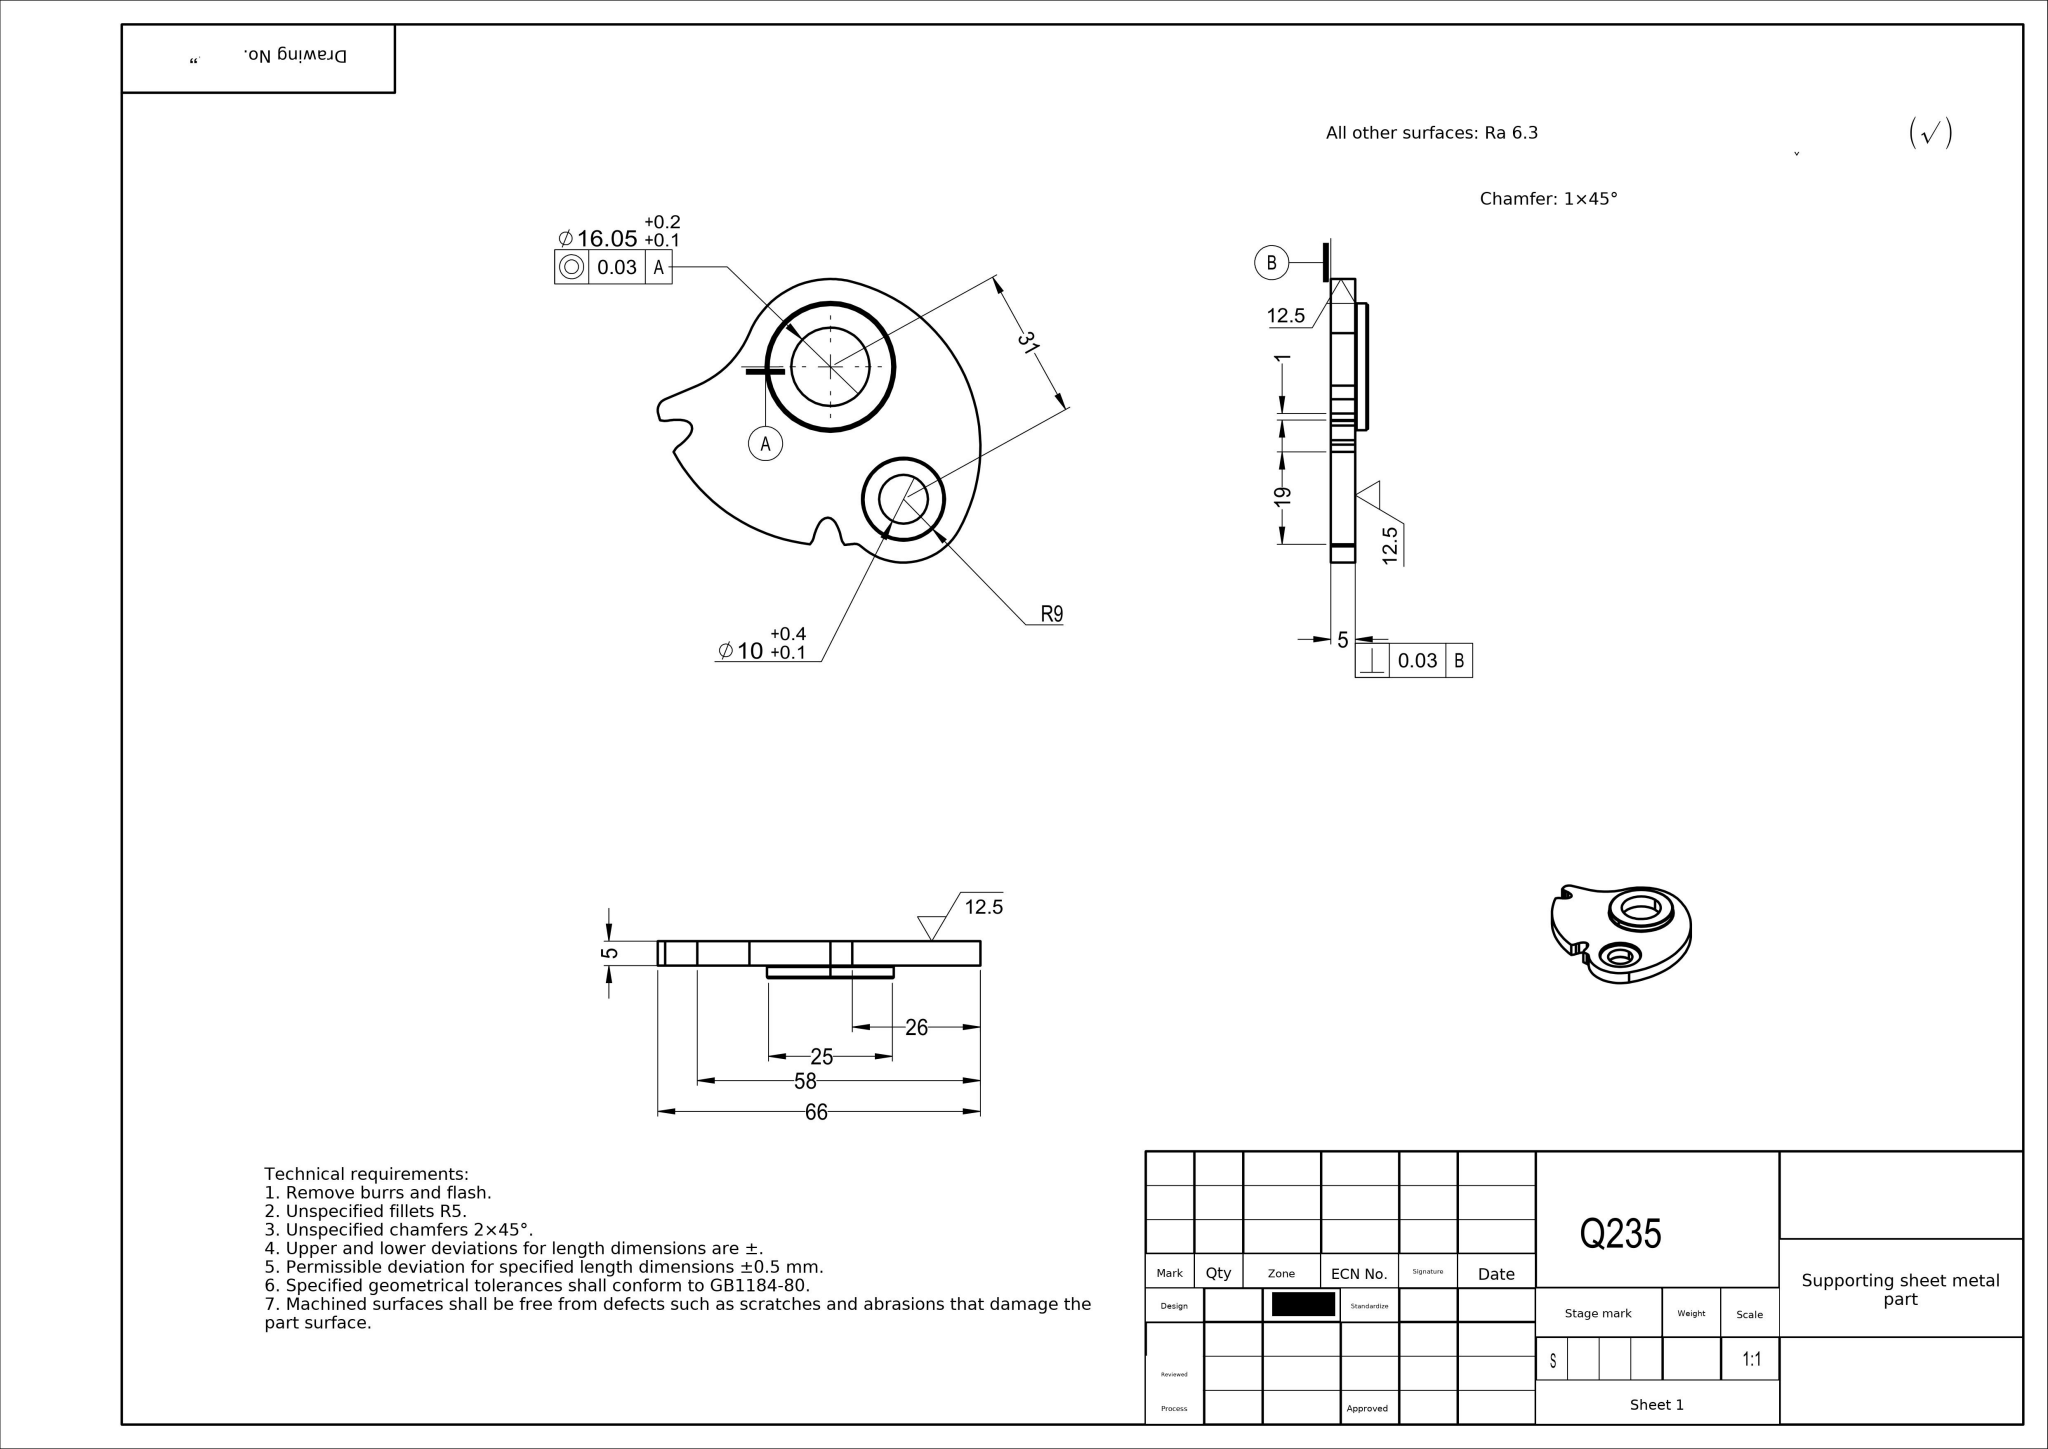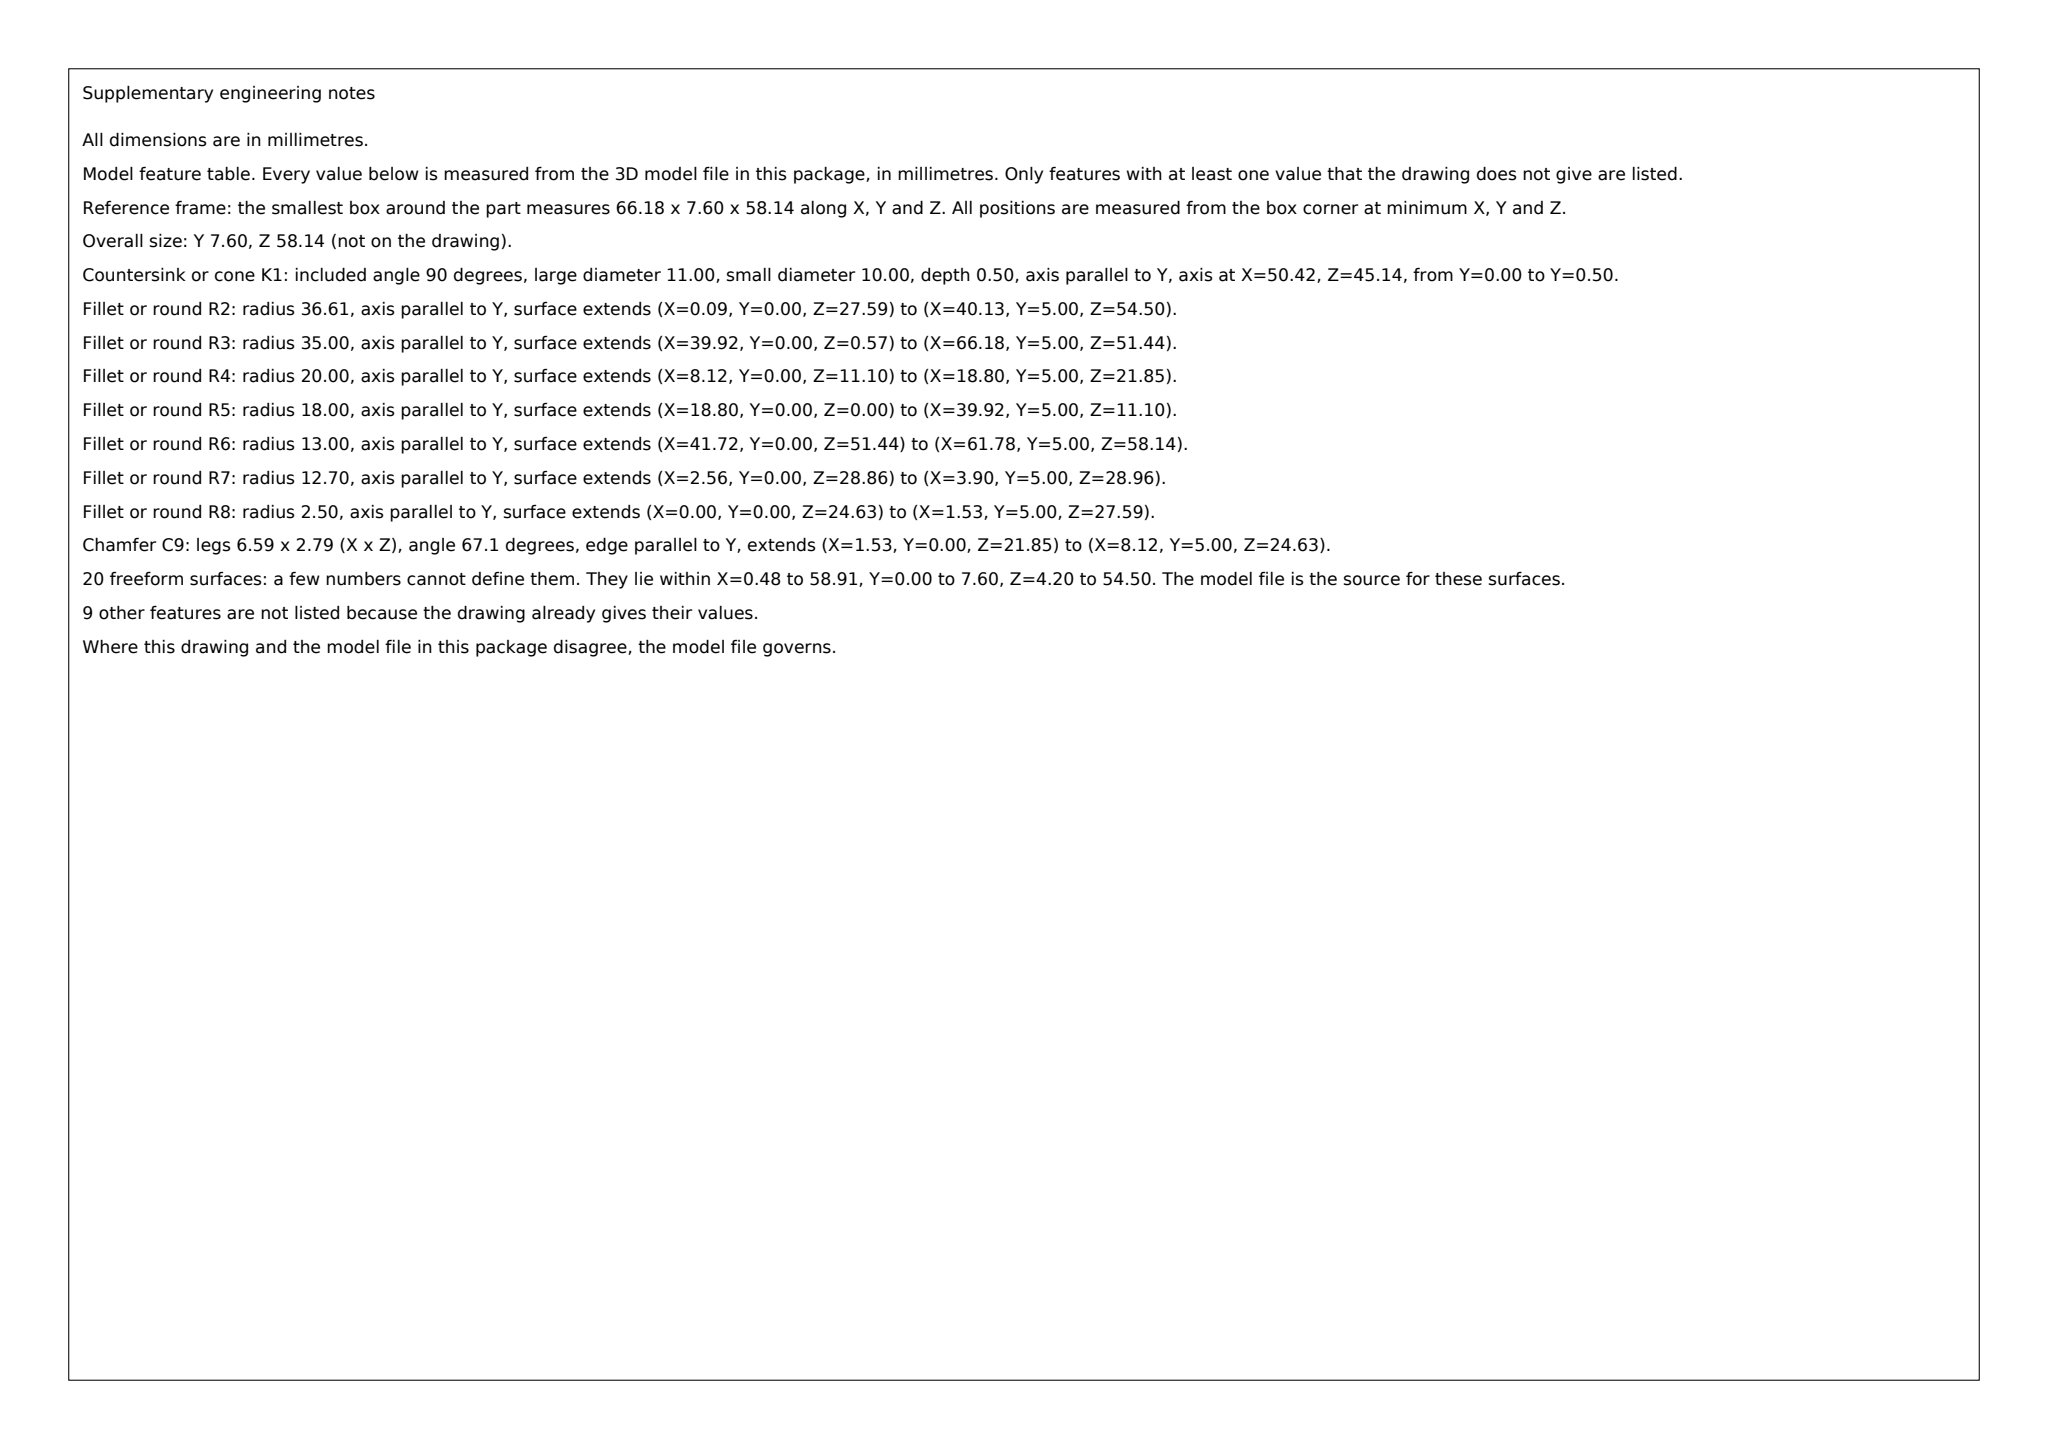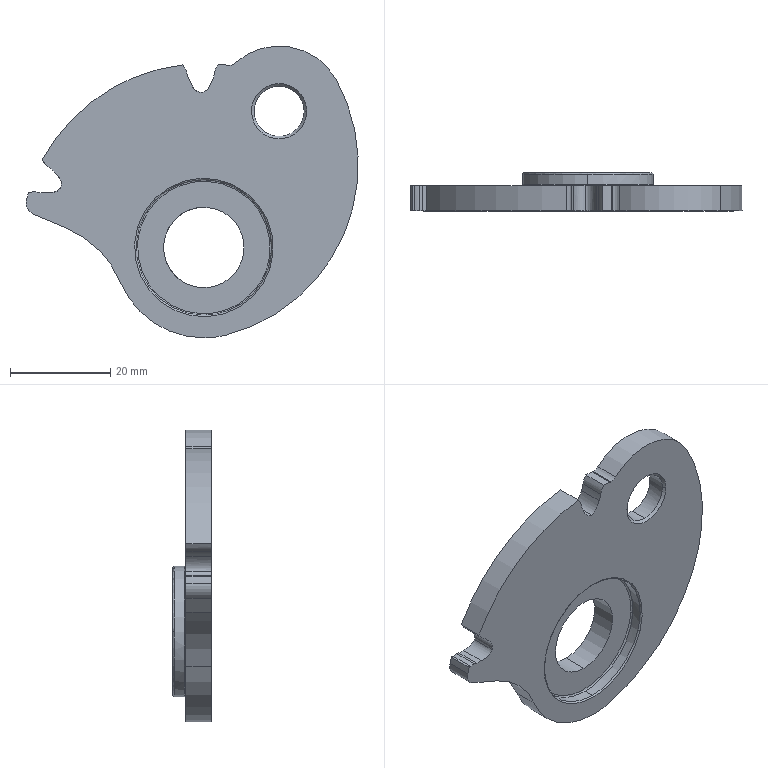Part | SolidWorks | mm | material Q235 | 1 solid | 53 faces | box 66.18 x 7.6 x 58.14 mm | volume 11489 mm3 | cylinder 25 | spline 20 | plane 6 | cone 2 | commonest cylinder face diameters 26 x3 73.228 x3 16.05 x2 27 x2 10 x2 17 x2 4 x2 36 x2